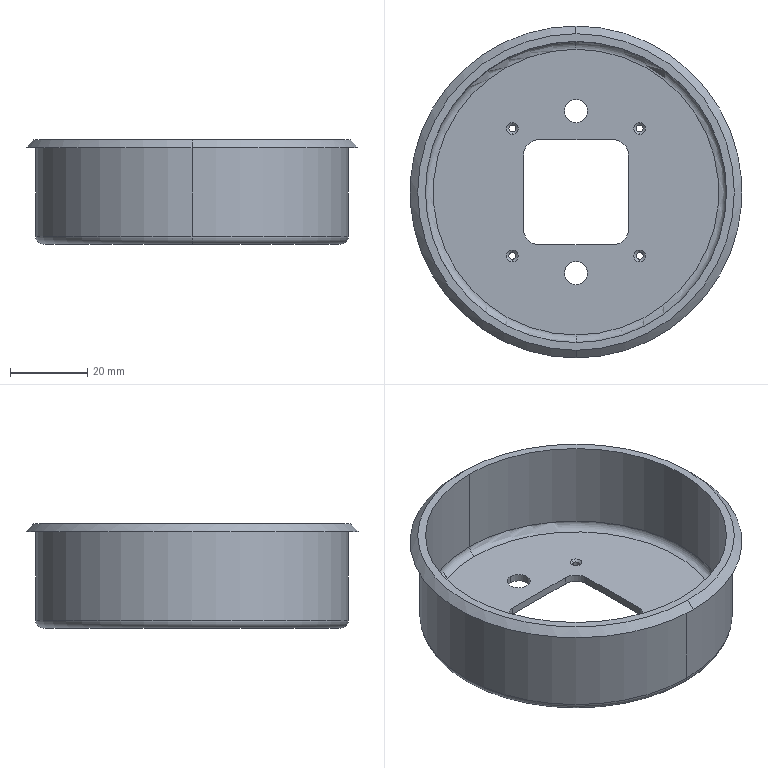Component | SolidWorks | GMotorCover2-1 | 1 solid | 42 faces | volume 18854 mm3 | cylinder 20 | cone 10 | plane 8 | torus 4 | commonest cylinder face diameters 1.778 x8 6 x4 8 x4 78 x2 81 x2